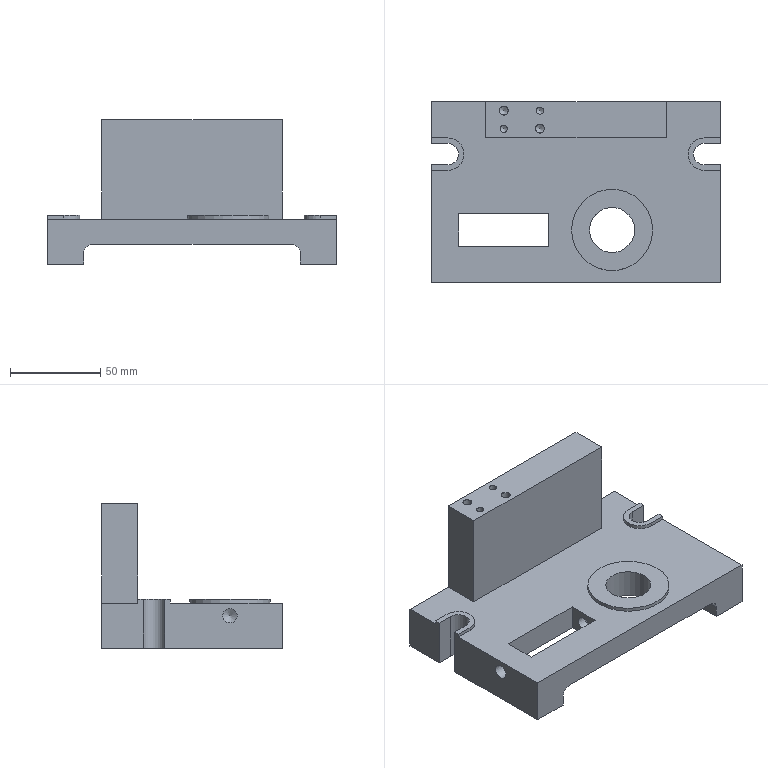Component | NX | FIXTURE_BODY | 1 solid | 54 faces | volume 350695 mm3 | plane 32 | cylinder 15 | cone 7 | commonest cylinder face diameters 10 x3 4 x2 4.826 x2 12 x2 18 x2 8 x2 25 x1 45 x1